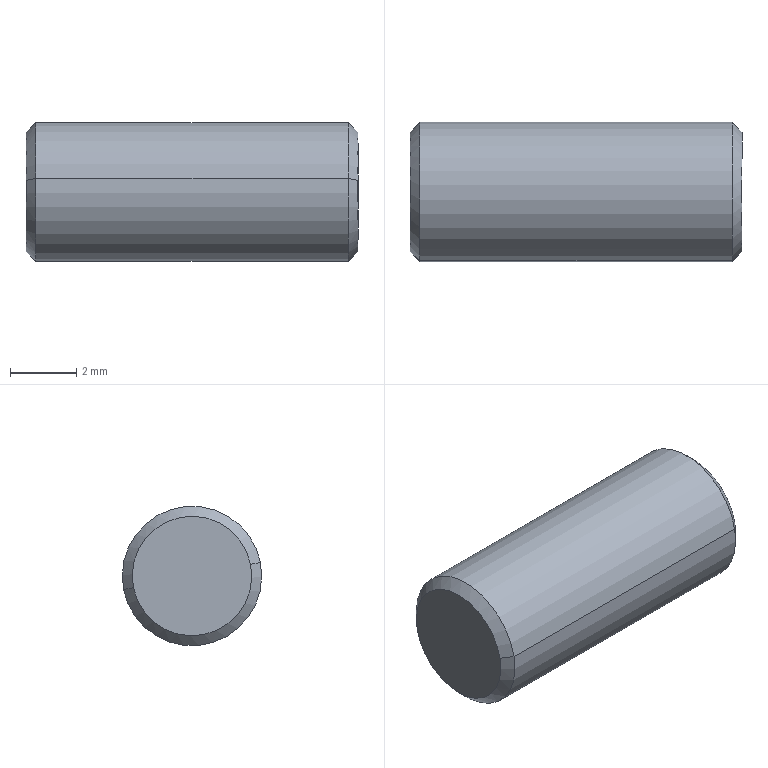Component | SolidWorks | M5SetScrew-2 | 1 solid | 15 faces | box 10 x 4.2 x 4.2 mm | volume 98 mm3 | plane 9 | cone 4 | cylinder 2 | commonest cylinder face diameters 4.2 x2 | material 45
STEP:
#1=COLOUR_RGB('',0.7922,0.8196,0.9333);
#2=FILL_AREA_STYLE_COLOUR('',#1);
#3=FILL_AREA_STYLE('',(#2));
#4=SURFACE_STYLE_FILL_AREA(#3);
#5=SURFACE_SIDE_STYLE('',(#4));
#6=SURFACE_STYLE_USAGE(.BOTH.,#5);
#7=PRESENTATION_STYLE_ASSIGNMENT((#6));
#8=CARTESIAN_POINT('',(0.5906,1.92,0.4586));
#9=VERTEX_POINT('',#8);
#10=CARTESIAN_POINT('',(0.5906,1.781,0.4863));
#11=VERTEX_POINT('',#10);
#12=CARTESIAN_POINT('',(0.5906,1.85,0.4724));
#13=DIRECTION('',(-1.,0.,0.));
#14=DIRECTION('',(-0.,-0.9807,0.1954));
#15=AXIS2_PLACEMENT_3D('',#12,#13,#14);
#16=CIRCLE('',#15,0.07087);
#17=EDGE_CURVE('',#9,#11,#16,.T.);
#18=ORIENTED_EDGE('',*,*,#17,.F.);
#19=CARTESIAN_POINT('',(0.6024,1.931,0.4563));
#20=VERTEX_POINT('',#19);
#21=CARTESIAN_POINT('',(0.6024,1.931,0.4563));
#22=DIRECTION('',(0.7071,0.6935,-0.1382));
#23=VECTOR('',#22,39.37);
#24=LINE('',#21,#23);
#25=EDGE_CURVE('',#9,#20,#24,.T.);
#26=ORIENTED_EDGE('',*,*,#25,.T.);
#27=CARTESIAN_POINT('',(0.6024,1.769,0.4886));
#28=VERTEX_POINT('',#27);
#29=CARTESIAN_POINT('',(0.6024,1.85,0.4724));
#30=DIRECTION('',(1.,-0.,-0.));
#31=DIRECTION('',(-0.,-0.9807,0.1954));
#32=AXIS2_PLACEMENT_3D('',#29,#30,#31);
#33=CIRCLE('',#32,0.08268);
#34=EDGE_CURVE('',#28,#20,#33,.T.);
#35=ORIENTED_EDGE('',*,*,#34,.F.);
#36=CARTESIAN_POINT('',(0.6024,1.769,0.4886));
#37=DIRECTION('',(0.7071,-0.6935,0.1382));
#38=VECTOR('',#37,39.37);
#39=LINE('',#36,#38);
#40=EDGE_CURVE('',#11,#28,#39,.T.);
#41=ORIENTED_EDGE('',*,*,#40,.F.);
#42=EDGE_LOOP('',(#18,#26,#35,#41));
#43=FACE_OUTER_BOUND('',#42,.T.);
#44=CARTESIAN_POINT('',(0.6024,1.85,0.4724));
#45=DIRECTION('',(1.,-0.,-0.));
#46=DIRECTION('',(-0.,-0.9807,0.1954));
#47=AXIS2_PLACEMENT_3D('',#44,#45,#46);
#48=CONICAL_SURFACE('',#47,0.08268,0.7854);
#49=ADVANCED_FACE('',(#43),#48,.T.);
#50=CARTESIAN_POINT('',(0.9843,1.781,0.4863));
#51=VERTEX_POINT('',#50);
#52=CARTESIAN_POINT('',(0.9843,1.92,0.4586));
#53=VERTEX_POINT('',#52);
#54=CARTESIAN_POINT('',(0.9843,1.85,0.4724));
#55=DIRECTION('',(1.,-0.,-0.));
#56=DIRECTION('',(-0.,-0.9807,0.1954));
#57=AXIS2_PLACEMENT_3D('',#54,#55,#56);
#58=CIRCLE('',#57,0.07087);
#59=EDGE_CURVE('',#51,#53,#58,.T.);
#60=ORIENTED_EDGE('',*,*,#59,.F.);
#61=CARTESIAN_POINT('',(0.9724,1.769,0.4886));
#62=VERTEX_POINT('',#61);
#63=CARTESIAN_POINT('',(0.9843,1.781,0.4863));
#64=DIRECTION('',(-0.7071,-0.6935,0.1382));
#65=VECTOR('',#64,39.37);
#66=LINE('',#63,#65);
#67=EDGE_CURVE('',#51,#62,#66,.T.);
#68=ORIENTED_EDGE('',*,*,#67,.T.);
#69=CARTESIAN_POINT('',(0.9724,1.931,0.4563));
#70=VERTEX_POINT('',#69);
#71=CARTESIAN_POINT('',(0.9724,1.85,0.4724));
#72=DIRECTION('',(-1.,0.,0.));
#73=DIRECTION('',(-0.,-0.9807,0.1954));
#74=AXIS2_PLACEMENT_3D('',#71,#72,#73);
#75=CIRCLE('',#74,0.08268);
#76=EDGE_CURVE('',#70,#62,#75,.T.);
#77=ORIENTED_EDGE('',*,*,#76,.F.);
#78=CARTESIAN_POINT('',(0.9843,1.92,0.4586));
#79=DIRECTION('',(-0.7071,0.6935,-0.1382));
#80=VECTOR('',#79,39.37);
#81=LINE('',#78,#80);
#82=EDGE_CURVE('',#53,#70,#81,.T.);
#83=ORIENTED_EDGE('',*,*,#82,.F.);
#84=EDGE_LOOP('',(#60,#68,#77,#83));
#85=FACE_OUTER_BOUND('',#84,.T.);
#86=CARTESIAN_POINT('',(0.9843,1.85,0.4724));
#87=DIRECTION('',(-1.,0.,0.));
#88=DIRECTION('',(0.,0.9807,-0.1954));
#89=AXIS2_PLACEMENT_3D('',#86,#87,#88);
#90=CONICAL_SURFACE('',#89,0.07087,0.7854);
#91=ADVANCED_FACE('',(#85),#90,.T.);
#92=ORIENTED_EDGE('',*,*,#76,.T.);
#93=CARTESIAN_POINT('',(0.9843,1.769,0.4886));
#94=DIRECTION('',(-1.,0.,0.));
#95=VECTOR('',#94,39.37);
#96=LINE('',#93,#95);
#97=EDGE_CURVE('',#62,#28,#96,.T.);
#98=ORIENTED_EDGE('',*,*,#97,.T.);
#99=ORIENTED_EDGE('',*,*,#34,.T.);
#100=CARTESIAN_POINT('',(0.9843,1.931,0.4563));
#101=DIRECTION('',(-1.,0.,0.));
#102=VECTOR('',#101,39.37);
#103=LINE('',#100,#102);
#104=EDGE_CURVE('',#70,#20,#103,.T.);
#105=ORIENTED_EDGE('',*,*,#104,.F.);
#106=EDGE_LOOP('',(#92,#98,#99,#105));
#107=FACE_OUTER_BOUND('',#106,.T.);
#108=CARTESIAN_POINT('',(0.9843,1.85,0.4724));
#109=DIRECTION('',(-1.,0.,0.));
#110=DIRECTION('',(0.,0.9807,-0.1954));
#111=AXIS2_PLACEMENT_3D('',#108,#109,#110);
#112=CYLINDRICAL_SURFACE('',#111,0.08268);
#113=ADVANCED_FACE('',(#107),#112,.T.);
#114=ORIENTED_EDGE('',*,*,#97,.F.);
#115=CARTESIAN_POINT('',(0.9724,1.85,0.4724));
#116=DIRECTION('',(-1.,0.,0.));
#117=DIRECTION('',(-0.,-0.9807,0.1954));
#118=AXIS2_PLACEMENT_3D('',#115,#116,#117);
#119=CIRCLE('',#118,0.08268);
#120=EDGE_CURVE('',#62,#70,#119,.T.);
#121=ORIENTED_EDGE('',*,*,#120,.T.);
#122=ORIENTED_EDGE('',*,*,#104,.T.);
#123=CARTESIAN_POINT('',(0.6024,1.85,0.4724));
#124=DIRECTION('',(1.,-0.,-0.));
#125=DIRECTION('',(-0.,-0.9807,0.1954));
#126=AXIS2_PLACEMENT_3D('',#123,#124,#125);
#127=CIRCLE('',#126,0.08268);
#128=EDGE_CURVE('',#20,#28,#127,.T.);
#129=ORIENTED_EDGE('',*,*,#128,.T.);
#130=EDGE_LOOP('',(#114,#121,#122,#129));
#131=FACE_OUTER_BOUND('',#130,.T.);
#132=CARTESIAN_POINT('',(0.9843,1.85,0.4724));
#133=DIRECTION('',(-1.,0.,0.));
#134=DIRECTION('',(0.,0.9807,-0.1954));
#135=AXIS2_PLACEMENT_3D('',#132,#133,#134);
#136=CYLINDRICAL_SURFACE('',#135,0.08268);
#137=ADVANCED_FACE('',(#131),#136,.T.);
#138=CARTESIAN_POINT('',(0.9843,1.828,0.537));
#139=VERTEX_POINT('',#138);
#140=CARTESIAN_POINT('',(0.9843,1.784,0.4858));
#141=VERTEX_POINT('',#140);
#142=CARTESIAN_POINT('',(0.9843,1.828,0.537));
#143=DIRECTION('',(-0.,-0.6596,-0.7516));
#144=VECTOR('',#143,39.37);
#145=LINE('',#142,#144);
#146=EDGE_CURVE('',#139,#141,#145,.T.);
#147=ORIENTED_EDGE('',*,*,#146,.F.);
#148=CARTESIAN_POINT('',(0.9843,1.895,0.5237));
#149=VERTEX_POINT('',#148);
#150=CARTESIAN_POINT('',(0.9843,1.895,0.5237));
#151=DIRECTION('',(-0.,-0.9807,0.1954));
#152=VECTOR('',#151,39.37);
#153=LINE('',#150,#152);
#154=EDGE_CURVE('',#149,#139,#153,.T.);
#155=ORIENTED_EDGE('',*,*,#154,.F.);
#156=CARTESIAN_POINT('',(0.9843,1.917,0.4591));
#157=VERTEX_POINT('',#156);
#158=CARTESIAN_POINT('',(0.9843,1.917,0.4591));
#159=DIRECTION('',(-0.,-0.3211,0.947));
#160=VECTOR('',#159,39.37);
#161=LINE('',#158,#160);
#162=EDGE_CURVE('',#157,#149,#161,.T.);
#163=ORIENTED_EDGE('',*,*,#162,.F.);
#164=CARTESIAN_POINT('',(0.9843,1.872,0.4079));
#165=VERTEX_POINT('',#164);
#166=CARTESIAN_POINT('',(0.9843,1.872,0.4079));
#167=DIRECTION('',(0.,0.6596,0.7516));
#168=VECTOR('',#167,39.37);
#169=LINE('',#166,#168);
#170=EDGE_CURVE('',#165,#157,#169,.T.);
#171=ORIENTED_EDGE('',*,*,#170,.F.);
#172=CARTESIAN_POINT('',(0.9843,1.805,0.4212));
#173=VERTEX_POINT('',#172);
#174=CARTESIAN_POINT('',(0.9843,1.805,0.4212));
#175=DIRECTION('',(0.,0.9807,-0.1954));
#176=VECTOR('',#175,39.37);
#177=LINE('',#174,#176);
#178=EDGE_CURVE('',#173,#165,#177,.T.);
#179=ORIENTED_EDGE('',*,*,#178,.F.);
#180=CARTESIAN_POINT('',(0.9843,1.784,0.4858));
#181=DIRECTION('',(0.,0.3211,-0.947));
#182=VECTOR('',#181,39.37);
#183=LINE('',#180,#182);
#184=EDGE_CURVE('',#141,#173,#183,.T.);
#185=ORIENTED_EDGE('',*,*,#184,.F.);
#186=EDGE_LOOP('',(#147,#155,#163,#171,#179,#185));
#187=FACE_BOUND('',#186,.T.);
#188=CARTESIAN_POINT('',(0.9843,1.85,0.4724));
#189=DIRECTION('',(1.,-0.,-0.));
#190=DIRECTION('',(-0.,-0.9807,0.1954));
#191=AXIS2_PLACEMENT_3D('',#188,#189,#190);
#192=CIRCLE('',#191,0.07087);
#193=EDGE_CURVE('',#53,#51,#192,.T.);
#194=ORIENTED_EDGE('',*,*,#193,.T.);
#195=ORIENTED_EDGE('',*,*,#59,.T.);
#196=EDGE_LOOP('',(#194,#195));
#197=FACE_OUTER_BOUND('',#196,.T.);
#198=CARTESIAN_POINT('',(0.9843,1.85,0.4724));
#199=DIRECTION('',(1.,-0.,-0.));
#200=DIRECTION('',(-0.,-0.9807,0.1954));
#201=AXIS2_PLACEMENT_3D('',#198,#199,#200);
#202=PLANE('',#201);
#203=ADVANCED_FACE('',(#187,#197),#202,.T.);
#204=CARTESIAN_POINT('',(0.5906,1.85,0.4724));
#205=DIRECTION('',(-1.,0.,0.));
#206=DIRECTION('',(-0.,-0.9807,0.1954));
#207=AXIS2_PLACEMENT_3D('',#204,#205,#206);
#208=CIRCLE('',#207,0.07087);
#209=EDGE_CURVE('',#11,#9,#208,.T.);
#210=ORIENTED_EDGE('',*,*,#209,.T.);
#211=ORIENTED_EDGE('',*,*,#17,.T.);
#212=EDGE_LOOP('',(#210,#211));
#213=FACE_OUTER_BOUND('',#212,.T.);
#214=CARTESIAN_POINT('',(0.5906,1.85,0.4724));
#215=DIRECTION('',(1.,-0.,-0.));
#216=DIRECTION('',(-0.,-0.9807,0.1954));
#217=AXIS2_PLACEMENT_3D('',#214,#215,#216);
#218=PLANE('',#217);
#219=ADVANCED_FACE('',(#213),#218,.F.);
#220=ORIENTED_EDGE('',*,*,#67,.F.);
#221=ORIENTED_EDGE('',*,*,#193,.F.);
#222=ORIENTED_EDGE('',*,*,#82,.T.);
#223=ORIENTED_EDGE('',*,*,#120,.F.);
#224=EDGE_LOOP('',(#220,#221,#222,#223));
#225=FACE_OUTER_BOUND('',#224,.T.);
#226=CARTESIAN_POINT('',(0.9843,1.85,0.4724));
#227=DIRECTION('',(-1.,0.,0.));
#228=DIRECTION('',(0.,0.9807,-0.1954));
#229=AXIS2_PLACEMENT_3D('',#226,#227,#228);
#230=CONICAL_SURFACE('',#229,0.07087,0.7854);
#231=ADVANCED_FACE('',(#225),#230,.T.);
#232=ORIENTED_EDGE('',*,*,#25,.F.);
#233=ORIENTED_EDGE('',*,*,#209,.F.);
#234=ORIENTED_EDGE('',*,*,#40,.T.);
#235=ORIENTED_EDGE('',*,*,#128,.F.);
#236=EDGE_LOOP('',(#232,#233,#234,#235));
#237=FACE_OUTER_BOUND('',#236,.T.);
#238=CARTESIAN_POINT('',(0.6024,1.85,0.4724));
#239=DIRECTION('',(1.,-0.,-0.));
#240=DIRECTION('',(-0.,-0.9807,0.1954));
#241=AXIS2_PLACEMENT_3D('',#238,#239,#240);
#242=CONICAL_SURFACE('',#241,0.08268,0.7854);
#243=ADVANCED_FACE('',(#237),#242,.T.);
#244=ORIENTED_EDGE('',*,*,#146,.T.);
#245=CARTESIAN_POINT('',(0.7874,1.784,0.4858));
#246=VERTEX_POINT('',#245);
#247=CARTESIAN_POINT('',(0.7874,1.784,0.4858));
#248=DIRECTION('',(1.,-0.,-0.));
#249=VECTOR('',#248,39.37);
#250=LINE('',#247,#249);
#251=EDGE_CURVE('',#246,#141,#250,.T.);
#252=ORIENTED_EDGE('',*,*,#251,.F.);
#253=CARTESIAN_POINT('',(0.7874,1.828,0.537));
#254=VERTEX_POINT('',#253);
#255=CARTESIAN_POINT('',(0.7874,1.828,0.537));
#256=DIRECTION('',(-0.,-0.6596,-0.7516));
#257=VECTOR('',#256,39.37);
#258=LINE('',#255,#257);
#259=EDGE_CURVE('',#254,#246,#258,.T.);
#260=ORIENTED_EDGE('',*,*,#259,.F.);
#261=CARTESIAN_POINT('',(0.7874,1.828,0.537));
#262=DIRECTION('',(1.,-0.,-0.));
#263=VECTOR('',#262,39.37);
#264=LINE('',#261,#263);
#265=EDGE_CURVE('',#254,#139,#264,.T.);
#266=ORIENTED_EDGE('',*,*,#265,.T.);
#267=EDGE_LOOP('',(#244,#252,#260,#266));
#268=FACE_OUTER_BOUND('',#267,.T.);
#269=CARTESIAN_POINT('',(0.7874,1.828,0.537));
#270=DIRECTION('',(-0.,-0.7516,0.6596));
#271=DIRECTION('',(-0.,-0.6596,-0.7516));
#272=AXIS2_PLACEMENT_3D('',#269,#270,#271);
#273=PLANE('',#272);
#274=ADVANCED_FACE('',(#268),#273,.F.);
#275=ORIENTED_EDGE('',*,*,#154,.T.);
#276=ORIENTED_EDGE('',*,*,#265,.F.);
#277=CARTESIAN_POINT('',(0.7874,1.895,0.5237));
#278=VERTEX_POINT('',#277);
#279=CARTESIAN_POINT('',(0.7874,1.895,0.5237));
#280=DIRECTION('',(-0.,-0.9807,0.1954));
#281=VECTOR('',#280,39.37);
#282=LINE('',#279,#281);
#283=EDGE_CURVE('',#278,#254,#282,.T.);
#284=ORIENTED_EDGE('',*,*,#283,.F.);
#285=CARTESIAN_POINT('',(0.7874,1.895,0.5237));
#286=DIRECTION('',(1.,-0.,-0.));
#287=VECTOR('',#286,39.37);
#288=LINE('',#285,#287);
#289=EDGE_CURVE('',#278,#149,#288,.T.);
#290=ORIENTED_EDGE('',*,*,#289,.T.);
#291=EDGE_LOOP('',(#275,#276,#284,#290));
#292=FACE_OUTER_BOUND('',#291,.T.);
#293=CARTESIAN_POINT('',(0.7874,1.895,0.5237));
#294=DIRECTION('',(0.,0.1954,0.9807));
#295=DIRECTION('',(-1.,0.,0.));
#296=AXIS2_PLACEMENT_3D('',#293,#294,#295);
#297=PLANE('',#296);
#298=ADVANCED_FACE('',(#292),#297,.F.);
#299=ORIENTED_EDGE('',*,*,#162,.T.);
#300=ORIENTED_EDGE('',*,*,#289,.F.);
#301=CARTESIAN_POINT('',(0.7874,1.917,0.4591));
#302=VERTEX_POINT('',#301);
#303=CARTESIAN_POINT('',(0.7874,1.917,0.4591));
#304=DIRECTION('',(-0.,-0.3211,0.947));
#305=VECTOR('',#304,39.37);
#306=LINE('',#303,#305);
#307=EDGE_CURVE('',#302,#278,#306,.T.);
#308=ORIENTED_EDGE('',*,*,#307,.F.);
#309=CARTESIAN_POINT('',(0.7874,1.917,0.4591));
#310=DIRECTION('',(1.,-0.,-0.));
#311=VECTOR('',#310,39.37);
#312=LINE('',#309,#311);
#313=EDGE_CURVE('',#302,#157,#312,.T.);
#314=ORIENTED_EDGE('',*,*,#313,.T.);
#315=EDGE_LOOP('',(#299,#300,#308,#314));
#316=FACE_OUTER_BOUND('',#315,.T.);
#317=CARTESIAN_POINT('',(0.7874,1.917,0.4591));
#318=DIRECTION('',(0.,0.947,0.3211));
#319=DIRECTION('',(-0.,-0.3211,0.947));
#320=AXIS2_PLACEMENT_3D('',#317,#318,#319);
#321=PLANE('',#320);
#322=ADVANCED_FACE('',(#316),#321,.F.);
#323=ORIENTED_EDGE('',*,*,#170,.T.);
#324=ORIENTED_EDGE('',*,*,#313,.F.);
#325=CARTESIAN_POINT('',(0.7874,1.872,0.4079));
#326=VERTEX_POINT('',#325);
#327=CARTESIAN_POINT('',(0.7874,1.872,0.4079));
#328=DIRECTION('',(0.,0.6596,0.7516));
#329=VECTOR('',#328,39.37);
#330=LINE('',#327,#329);
#331=EDGE_CURVE('',#326,#302,#330,.T.);
#332=ORIENTED_EDGE('',*,*,#331,.F.);
#333=CARTESIAN_POINT('',(0.7874,1.872,0.4079));
#334=DIRECTION('',(1.,-0.,-0.));
#335=VECTOR('',#334,39.37);
#336=LINE('',#333,#335);
#337=EDGE_CURVE('',#326,#165,#336,.T.);
#338=ORIENTED_EDGE('',*,*,#337,.T.);
#339=EDGE_LOOP('',(#323,#324,#332,#338));
#340=FACE_OUTER_BOUND('',#339,.T.);
#341=CARTESIAN_POINT('',(0.7874,1.872,0.4079));
#342=DIRECTION('',(0.,0.7516,-0.6596));
#343=DIRECTION('',(0.,0.6596,0.7516));
#344=AXIS2_PLACEMENT_3D('',#341,#342,#343);
#345=PLANE('',#344);
#346=ADVANCED_FACE('',(#340),#345,.F.);
#347=ORIENTED_EDGE('',*,*,#178,.T.);
#348=ORIENTED_EDGE('',*,*,#337,.F.);
#349=CARTESIAN_POINT('',(0.7874,1.805,0.4212));
#350=VERTEX_POINT('',#349);
#351=CARTESIAN_POINT('',(0.7874,1.805,0.4212));
#352=DIRECTION('',(0.,0.9807,-0.1954));
#353=VECTOR('',#352,39.37);
#354=LINE('',#351,#353);
#355=EDGE_CURVE('',#350,#326,#354,.T.);
#356=ORIENTED_EDGE('',*,*,#355,.F.);
#357=CARTESIAN_POINT('',(0.7874,1.805,0.4212));
#358=DIRECTION('',(1.,-0.,-0.));
#359=VECTOR('',#358,39.37);
#360=LINE('',#357,#359);
#361=EDGE_CURVE('',#350,#173,#360,.T.);
#362=ORIENTED_EDGE('',*,*,#361,.T.);
#363=EDGE_LOOP('',(#347,#348,#356,#362));
#364=FACE_OUTER_BOUND('',#363,.T.);
#365=CARTESIAN_POINT('',(0.7874,1.805,0.4212));
#366=DIRECTION('',(-0.,-0.1954,-0.9807));
#367=DIRECTION('',(1.,-0.,-0.));
#368=AXIS2_PLACEMENT_3D('',#365,#366,#367);
#369=PLANE('',#368);
#370=ADVANCED_FACE('',(#364),#369,.F.);
#371=ORIENTED_EDGE('',*,*,#184,.T.);
#372=ORIENTED_EDGE('',*,*,#361,.F.);
#373=CARTESIAN_POINT('',(0.7874,1.784,0.4858));
#374=DIRECTION('',(0.,0.3211,-0.947));
#375=VECTOR('',#374,39.37);
#376=LINE('',#373,#375);
#377=EDGE_CURVE('',#246,#350,#376,.T.);
#378=ORIENTED_EDGE('',*,*,#377,.F.);
#379=ORIENTED_EDGE('',*,*,#251,.T.);
#380=EDGE_LOOP('',(#371,#372,#378,#379));
#381=FACE_OUTER_BOUND('',#380,.T.);
#382=CARTESIAN_POINT('',(0.7874,1.784,0.4858));
#383=DIRECTION('',(-0.,-0.947,-0.3211));
#384=DIRECTION('',(0.,0.3211,-0.947));
#385=AXIS2_PLACEMENT_3D('',#382,#383,#384);
#386=PLANE('',#385);
#387=ADVANCED_FACE('',(#381),#386,.F.);
#388=ORIENTED_EDGE('',*,*,#259,.T.);
#389=ORIENTED_EDGE('',*,*,#377,.T.);
#390=ORIENTED_EDGE('',*,*,#355,.T.);
#391=ORIENTED_EDGE('',*,*,#331,.T.);
#392=ORIENTED_EDGE('',*,*,#307,.T.);
#393=ORIENTED_EDGE('',*,*,#283,.T.);
#394=EDGE_LOOP('',(#388,#389,#390,#391,#392,#393));
#395=FACE_OUTER_BOUND('',#394,.T.);
#396=CARTESIAN_POINT('',(0.7874,1.85,0.4724));
#397=DIRECTION('',(1.,-0.,-0.));
#398=DIRECTION('',(-0.,-0.9807,0.1954));
#399=AXIS2_PLACEMENT_3D('',#396,#397,#398);
#400=PLANE('',#399);
#401=ADVANCED_FACE('',(#395),#400,.T.);
#402=CLOSED_SHELL('',(#49,#91,#113,#137,#203,#219,#231,#243,#274,#298,#322,#346,#370,#387,#401));
#403=MANIFOLD_SOLID_BREP('',#402);
#404=STYLED_ITEM('',(#7),#403);
#405=PRESENTATION_LAYER_ASSIGNMENT('','',(#404));
#406=(LENGTH_UNIT()NAMED_UNIT(*)SI_UNIT($,.METRE.));
#407=LENGTH_MEASURE_WITH_UNIT(LENGTH_MEASURE(0.0254),#406);
#408=DIMENSIONAL_EXPONENTS(1.,0.,0.,0.,0.,0.,0.);
#409=(CONVERSION_BASED_UNIT('',#407)LENGTH_UNIT()NAMED_UNIT(#408));
#410=UNCERTAINTY_MEASURE_WITH_UNIT(LENGTH_MEASURE(0.00001),#409,'','');
#411=(NAMED_UNIT(*)PLANE_ANGLE_UNIT()SI_UNIT($,.RADIAN.));
#412=(NAMED_UNIT(*)SI_UNIT($,.STERADIAN.)SOLID_ANGLE_UNIT());
#413=(GEOMETRIC_REPRESENTATION_CONTEXT(3)GLOBAL_UNCERTAINTY_ASSIGNED_CONTEXT((#410))GLOBAL_UNIT_ASSIGNED_CONTEXT((#409,#411,#412))REPRESENTATION_CONTEXT('',''));
#414=MECHANICAL_DESIGN_GEOMETRIC_PRESENTATION_REPRESENTATION('',(#404),#413);
#415=CARTESIAN_POINT('',(0.,0.,0.));
#416=DIRECTION('',(0.,0.,1.));
#417=DIRECTION('',(1.,0.,0.));
#418=AXIS2_PLACEMENT_3D('',#415,#416,#417);
#419=(LENGTH_UNIT()NAMED_UNIT(*)SI_UNIT($,.METRE.));
#420=LENGTH_MEASURE_WITH_UNIT(LENGTH_MEASURE(0.0254),#419);
#421=DIMENSIONAL_EXPONENTS(1.,0.,0.,0.,0.,0.,0.);
#422=(CONVERSION_BASED_UNIT('',#420)LENGTH_UNIT()NAMED_UNIT(#421));
#423=UNCERTAINTY_MEASURE_WITH_UNIT(LENGTH_MEASURE(0.00001),#422,'','');
#424=(NAMED_UNIT(*)PLANE_ANGLE_UNIT()SI_UNIT($,.RADIAN.));
#425=(NAMED_UNIT(*)SI_UNIT($,.STERADIAN.)SOLID_ANGLE_UNIT());
#426=(GEOMETRIC_REPRESENTATION_CONTEXT(3)GLOBAL_UNCERTAINTY_ASSIGNED_CONTEXT((#423))GLOBAL_UNIT_ASSIGNED_CONTEXT((#422,#424,#425))REPRESENTATION_CONTEXT('',''));
#427=ADVANCED_BREP_SHAPE_REPRESENTATION('',(#403,#418),#426);